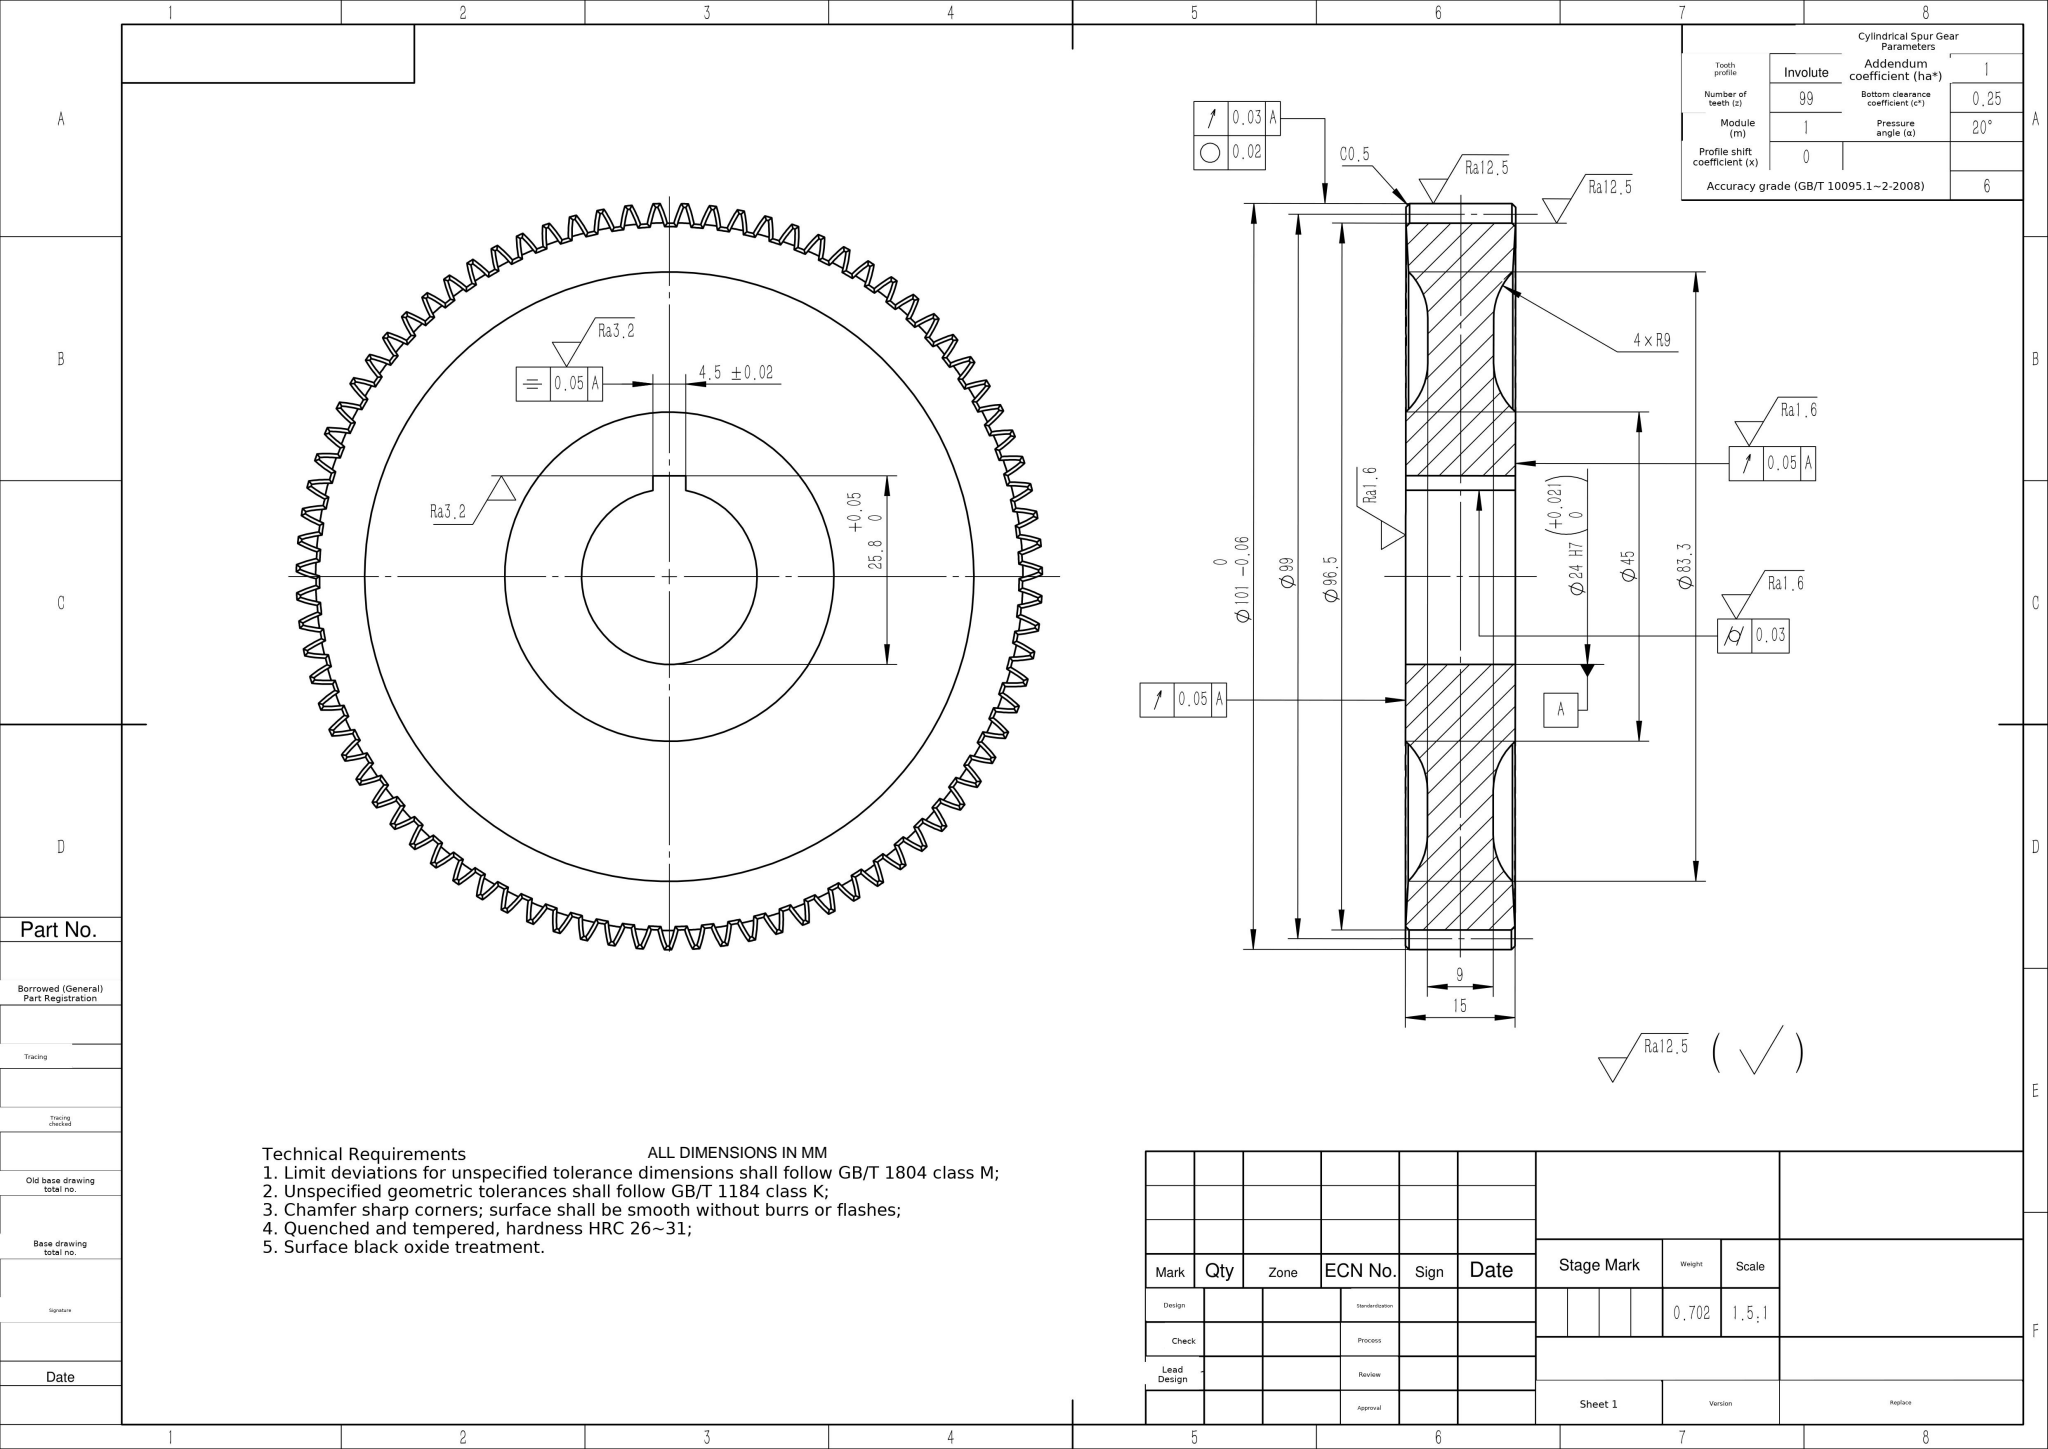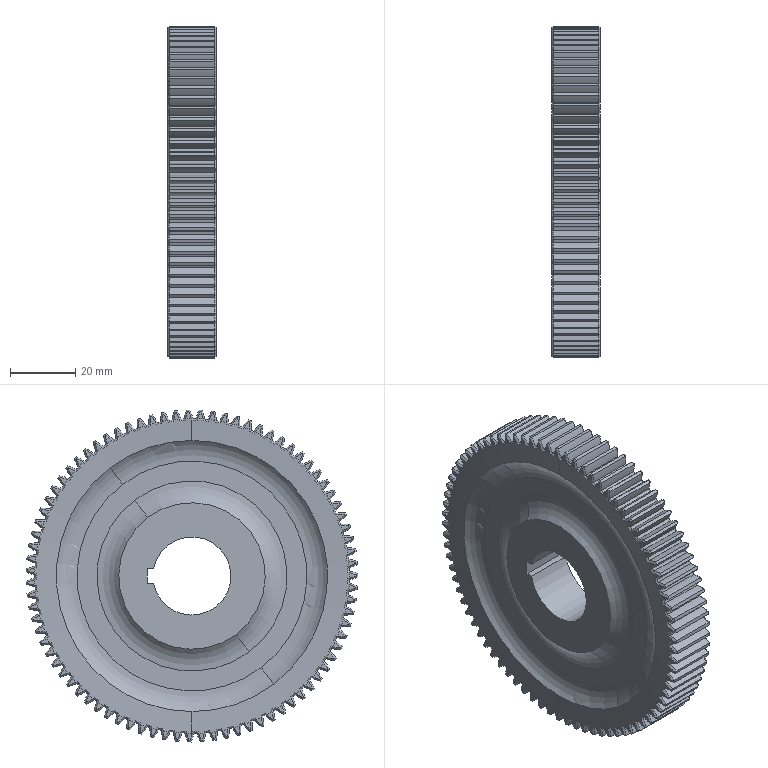Part | SolidWorks | mm | 1 solid | 1195 faces | box 15 x 101.98 x 101.99 mm | volume 90043 mm3 | cone 679 | cylinder 335 | plane 173 | torus 8 | commonest cylinder face diameters 32.65 x166 102 x83 96.6 x83 24 x3